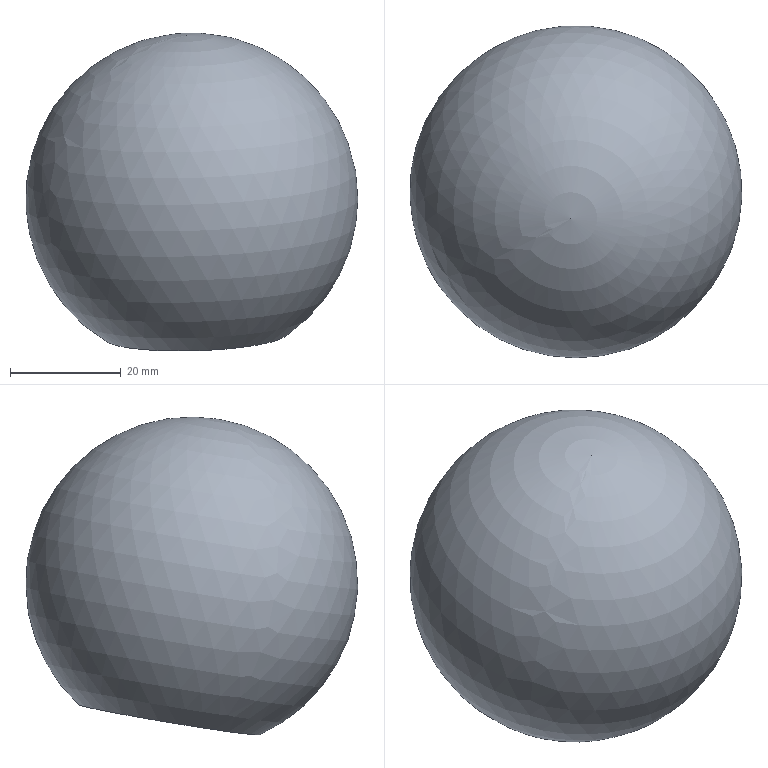Component | NX | HANDLE_KNOB | 1 solid | 5 faces | box 60 x 60 x 57.42 mm | volume 107862 mm3 | cone 2 | plane 1 | sphere 1 | cylinder 1 | commonest cylinder face diameters 14 x1
STEP:
#1=CARTESIAN_POINT('',(0.,0.,0.));
#2=DIRECTION('',(0.,0.,1.));
#3=DIRECTION('',(1.,0.,0.));
#4=AXIS2_PLACEMENT_3D('',#1,#2,#3);
#5=CARTESIAN_POINT('',(287.614,-214.929,616.056));
#6=VERTEX_POINT('',#5);
#7=CARTESIAN_POINT('',(283.581,-208.095,617.07));
#8=DIRECTION('',(-0.03071,-0.1644,0.9859));
#9=DIRECTION('',(0.5041,-0.8543,-0.1268));
#10=AXIS2_PLACEMENT_3D('',#7,#8,#9);
#11=CIRCLE('',#10,8.);
#12=CARTESIAN_POINT('',(283.581,-208.095,617.07));
#13=DIRECTION('',(-0.03071,-0.1644,0.9859));
#14=DIRECTION('',(0.5041,-0.8543,-0.1268));
#15=AXIS2_PLACEMENT_3D('',#12,#13,#14);
#16=PLANE('',#15);
#17=CARTESIAN_POINT('',(0.,0.));
#18=DIRECTION('',(1.,-0.));
#19=AXIS2_PLACEMENT_2D('',#17,#18);
#20=CIRCLE('',#19,8.);
#21=(GEOMETRIC_REPRESENTATION_CONTEXT(2)PARAMETRIC_REPRESENTATION_CONTEXT()REPRESENTATION_CONTEXT('',''));
#22=DEFINITIONAL_REPRESENTATION('',(#20),#21);
#23=PCURVE('',#16,#22);
#24=CARTESIAN_POINT('',(283.581,-208.095,617.07));
#25=DIRECTION('',(0.03071,0.1644,-0.9859));
#26=DIRECTION('',(-0.5041,0.8543,0.1268));
#27=AXIS2_PLACEMENT_3D('',#24,#25,#26);
#28=CONICAL_SURFACE('',#27,8.,0.7854);
#29=CARTESIAN_POINT('',(9.425,0.));
#30=DIRECTION('',(-1.,0.));
#31=VECTOR('',#30,1.);
#32=LINE('',#29,#31);
#33=(GEOMETRIC_REPRESENTATION_CONTEXT(2)PARAMETRIC_REPRESENTATION_CONTEXT()REPRESENTATION_CONTEXT('',''));
#34=DEFINITIONAL_REPRESENTATION('',(#32),#33);
#35=PCURVE('',#28,#34);
#36=SURFACE_CURVE('',#11,(#23,#35),.PCURVE_S1.);
#37=EDGE_CURVE('',#6,#6,#36,.T.);
#38=ORIENTED_EDGE('',*,*,#37,.T.);
#39=EDGE_LOOP('',(#38));
#40=FACE_BOUND('',#39,.T.);
#41=CARTESIAN_POINT('',(291.94,-222.262,614.968));
#42=VERTEX_POINT('',#41);
#43=CARTESIAN_POINT('',(269.268,-216.271,615.261));
#44=VERTEX_POINT('',#43);
#45=CARTESIAN_POINT('',(283.581,-208.095,617.07));
#46=DIRECTION('',(-0.03071,-0.1644,0.9859));
#47=DIRECTION('',(0.5041,-0.8543,-0.1268));
#48=AXIS2_PLACEMENT_3D('',#45,#46,#47);
#49=CIRCLE('',#48,16.583);
#50=CARTESIAN_POINT('',(0.,0.));
#51=DIRECTION('',(1.,0.));
#52=AXIS2_PLACEMENT_2D('',#50,#51);
#53=CIRCLE('',#52,16.583);
#54=(GEOMETRIC_REPRESENTATION_CONTEXT(2)PARAMETRIC_REPRESENTATION_CONTEXT()REPRESENTATION_CONTEXT('',''));
#55=DEFINITIONAL_REPRESENTATION('',(#53),#54);
#56=PCURVE('',#16,#55);
#57=CARTESIAN_POINT('',(282.813,-212.205,641.718));
#58=DIRECTION('',(-0.03071,-0.1644,0.9859));
#59=DIRECTION('',(-0.8631,-0.4931,-0.1091));
#60=AXIS2_PLACEMENT_3D('',#57,#58,#59);
#61=SPHERICAL_SURFACE('',#60,30.);
#62=CARTESIAN_POINT('',(1.571,-0.9851));
#63=CARTESIAN_POINT('',(1.666,-0.9851));
#64=CARTESIAN_POINT('',(1.856,-0.9851));
#65=CARTESIAN_POINT('',(2.142,-0.9851));
#66=CARTESIAN_POINT('',(2.428,-0.9851));
#67=CARTESIAN_POINT('',(2.713,-0.9851));
#68=CARTESIAN_POINT('',(2.999,-0.9851));
#69=CARTESIAN_POINT('',(3.284,-0.9851));
#70=CARTESIAN_POINT('',(3.57,-0.9851));
#71=CARTESIAN_POINT('',(3.856,-0.9851));
#72=CARTESIAN_POINT('',(4.141,-0.9851));
#73=CARTESIAN_POINT('',(4.427,-0.9851));
#74=CARTESIAN_POINT('',(4.712,-0.9851));
#75=CARTESIAN_POINT('',(4.998,-0.9851));
#76=CARTESIAN_POINT('',(5.284,-0.9851));
#77=CARTESIAN_POINT('',(5.569,-0.9851));
#78=CARTESIAN_POINT('',(5.855,-0.9851));
#79=CARTESIAN_POINT('',(6.14,-0.9851));
#80=CARTESIAN_POINT('',(6.426,-0.9851));
#81=CARTESIAN_POINT('',(6.712,-0.9851));
#82=CARTESIAN_POINT('',(6.997,-0.9851));
#83=CARTESIAN_POINT('',(7.283,-0.9851));
#84=CARTESIAN_POINT('',(7.568,-0.9851));
#85=CARTESIAN_POINT('',(7.759,-0.9851));
#86=CARTESIAN_POINT('',(7.854,-0.9851));
#87=B_SPLINE_CURVE_WITH_KNOTS('',3,(#62,#63,#64,#65,#66,#67,#68,#69,#70,#71,#72,#73,#74,#75,#76,#77,#78,#79,#80,#81,#82,#83,#84,#85,#86),.UNSPECIFIED.,.F.,.F.,(4,1,1,1,1,1,1,1,1,1,1,1,1,1,1,1,1,1,1,1,1,1,4),(0.,0.2856,0.5712,0.8568,1.142,1.428,1.714,1.999,2.285,2.57,2.856,3.142,3.427,3.713,3.998,4.284,4.57,4.855,5.141,5.426,5.712,5.998,6.283),.QUASI_UNIFORM_KNOTS.);
#88=(GEOMETRIC_REPRESENTATION_CONTEXT(2)PARAMETRIC_REPRESENTATION_CONTEXT()REPRESENTATION_CONTEXT('',''));
#89=DEFINITIONAL_REPRESENTATION('',(#87),#88);
#90=PCURVE('',#61,#89);
#91=SURFACE_CURVE('',#49,(#56,#90),.PCURVE_S1.);
#92=EDGE_CURVE('',#42,#44,#91,.T.);
#93=ORIENTED_EDGE('',*,*,#92,.F.);
#94=CARTESIAN_POINT('',(283.581,-208.095,617.07));
#95=DIRECTION('',(-0.03071,-0.1644,0.9859));
#96=DIRECTION('',(0.5041,-0.8543,-0.1268));
#97=AXIS2_PLACEMENT_3D('',#94,#95,#96);
#98=CIRCLE('',#97,16.583);
#99=CARTESIAN_POINT('',(0.,0.));
#100=DIRECTION('',(1.,0.));
#101=AXIS2_PLACEMENT_2D('',#99,#100);
#102=CIRCLE('',#101,16.583);
#103=(GEOMETRIC_REPRESENTATION_CONTEXT(2)PARAMETRIC_REPRESENTATION_CONTEXT()REPRESENTATION_CONTEXT('',''));
#104=DEFINITIONAL_REPRESENTATION('',(#102),#103);
#105=PCURVE('',#16,#104);
#106=CARTESIAN_POINT('',(-4.712,-0.9851));
#107=CARTESIAN_POINT('',(-4.617,-0.9851));
#108=CARTESIAN_POINT('',(-4.427,-0.9851));
#109=CARTESIAN_POINT('',(-4.141,-0.9851));
#110=CARTESIAN_POINT('',(-3.856,-0.9851));
#111=CARTESIAN_POINT('',(-3.57,-0.9851));
#112=CARTESIAN_POINT('',(-3.284,-0.9851));
#113=CARTESIAN_POINT('',(-2.999,-0.9851));
#114=CARTESIAN_POINT('',(-2.713,-0.9851));
#115=CARTESIAN_POINT('',(-2.428,-0.9851));
#116=CARTESIAN_POINT('',(-2.142,-0.9851));
#117=CARTESIAN_POINT('',(-1.856,-0.9851));
#118=CARTESIAN_POINT('',(-1.571,-0.9851));
#119=CARTESIAN_POINT('',(-1.285,-0.9851));
#120=CARTESIAN_POINT('',(-0.9996,-0.9851));
#121=CARTESIAN_POINT('',(-0.714,-0.9851));
#122=CARTESIAN_POINT('',(-0.4284,-0.9851));
#123=CARTESIAN_POINT('',(-0.1428,-0.9851));
#124=CARTESIAN_POINT('',(0.1428,-0.9851));
#125=CARTESIAN_POINT('',(0.4284,-0.9851));
#126=CARTESIAN_POINT('',(0.714,-0.9851));
#127=CARTESIAN_POINT('',(0.9996,-0.9851));
#128=CARTESIAN_POINT('',(1.285,-0.9851));
#129=CARTESIAN_POINT('',(1.476,-0.9851));
#130=CARTESIAN_POINT('',(1.571,-0.9851));
#131=B_SPLINE_CURVE_WITH_KNOTS('',3,(#106,#107,#108,#109,#110,#111,#112,#113,#114,#115,#116,#117,#118,#119,#120,#121,#122,#123,#124,#125,#126,#127,#128,#129,#130),.UNSPECIFIED.,.F.,.F.,(4,1,1,1,1,1,1,1,1,1,1,1,1,1,1,1,1,1,1,1,1,1,4),(0.,0.2856,0.5712,0.8568,1.142,1.428,1.714,1.999,2.285,2.57,2.856,3.142,3.427,3.713,3.998,4.284,4.57,4.855,5.141,5.426,5.712,5.998,6.283),.QUASI_UNIFORM_KNOTS.);
#132=(GEOMETRIC_REPRESENTATION_CONTEXT(2)PARAMETRIC_REPRESENTATION_CONTEXT()REPRESENTATION_CONTEXT('',''));
#133=DEFINITIONAL_REPRESENTATION('',(#131),#132);
#134=PCURVE('',#61,#133);
#135=SURFACE_CURVE('',#98,(#105,#134),.PCURVE_S1.);
#136=EDGE_CURVE('',#44,#42,#135,.T.);
#137=ORIENTED_EDGE('',*,*,#136,.F.);
#138=EDGE_LOOP('',(#93,#137));
#139=FACE_BOUND('',#138,.T.);
#140=ADVANCED_FACE('',(#40,#139),#16,.F.);
#141=ORIENTED_EDGE('',*,*,#92,.T.);
#142=CARTESIAN_POINT('',(281.892,-217.137,671.296));
#143=VERTEX_POINT('',#142);
#144=CARTESIAN_POINT('',(269.268,-216.271,615.261));
#145=CARTESIAN_POINT('',(262.211,-221.081,619.613));
#146=CARTESIAN_POINT('',(256.735,-225.416,627.052));
#147=CARTESIAN_POINT('',(253.936,-228.528,636.898));
#148=CARTESIAN_POINT('',(254.569,-229.774,647.81));
#149=CARTESIAN_POINT('',(258.684,-228.853,657.971));
#150=CARTESIAN_POINT('',(265.454,-226.013,665.754));
#151=CARTESIAN_POINT('',(273.619,-221.863,670.25));
#152=CARTESIAN_POINT('',(281.892,-217.137,671.296));
#153=B_SPLINE_CURVE_WITH_KNOTS('',8,(#144,#145,#146,#147,#148,#149,#150,#151,#152),.UNSPECIFIED.,.F.,.F.,(9,9),(-0.9851,1.571),.PIECEWISE_BEZIER_KNOTS.);
#154=CARTESIAN_POINT('',(6.283,0.));
#155=DIRECTION('',(0.,1.));
#156=VECTOR('',#155,1.);
#157=LINE('',#154,#156);
#158=(GEOMETRIC_REPRESENTATION_CONTEXT(2)PARAMETRIC_REPRESENTATION_CONTEXT()REPRESENTATION_CONTEXT('',''));
#159=DEFINITIONAL_REPRESENTATION('',(#157),#158);
#160=PCURVE('',#61,#159);
#161=CARTESIAN_POINT('',(0.,0.));
#162=DIRECTION('',(0.,1.));
#163=VECTOR('',#162,1.);
#164=LINE('',#161,#163);
#165=(GEOMETRIC_REPRESENTATION_CONTEXT(2)PARAMETRIC_REPRESENTATION_CONTEXT()REPRESENTATION_CONTEXT('',''));
#166=DEFINITIONAL_REPRESENTATION('',(#164),#165);
#167=PCURVE('',#61,#166);
#168=SEAM_CURVE('',#153,(#160,#167),.PCURVE_S1.);
#169=EDGE_CURVE('',#44,#143,#168,.T.);
#170=ORIENTED_EDGE('',*,*,#169,.T.);
#171=ORIENTED_EDGE('',*,*,#169,.F.);
#172=ORIENTED_EDGE('',*,*,#136,.T.);
#173=EDGE_LOOP('',(#141,#170,#171,#172));
#174=FACE_BOUND('',#173,.T.);
#175=ADVANCED_FACE('',(#174),#61,.T.);
#176=CARTESIAN_POINT('',(279.5,-205.074,635.704));
#177=VERTEX_POINT('',#176);
#178=CARTESIAN_POINT('',(286.557,-217.034,633.929));
#179=VERTEX_POINT('',#178);
#180=CARTESIAN_POINT('',(283.028,-211.054,634.817));
#181=DIRECTION('',(0.03071,0.1644,-0.9859));
#182=DIRECTION('',(0.5041,-0.8543,-0.1268));
#183=AXIS2_PLACEMENT_3D('',#180,#181,#182);
#184=CIRCLE('',#183,7.);
#185=CARTESIAN_POINT('',(283.028,-211.054,634.817));
#186=DIRECTION('',(0.03071,0.1644,-0.9859));
#187=DIRECTION('',(-0.5041,0.8543,0.1268));
#188=AXIS2_PLACEMENT_3D('',#185,#186,#187);
#189=CONICAL_SURFACE('',#188,7.,1.03);
#190=CARTESIAN_POINT('',(-3.142,0.));
#191=DIRECTION('',(1.,0.));
#192=VECTOR('',#191,1.);
#193=LINE('',#190,#192);
#194=(GEOMETRIC_REPRESENTATION_CONTEXT(2)PARAMETRIC_REPRESENTATION_CONTEXT()REPRESENTATION_CONTEXT('',''));
#195=DEFINITIONAL_REPRESENTATION('',(#193),#194);
#196=PCURVE('',#189,#195);
#197=CARTESIAN_POINT('',(283.581,-208.095,617.07));
#198=DIRECTION('',(-0.03071,-0.1644,0.9859));
#199=DIRECTION('',(0.5041,-0.8543,-0.1268));
#200=AXIS2_PLACEMENT_3D('',#197,#198,#199);
#201=CYLINDRICAL_SURFACE('',#200,7.);
#202=CARTESIAN_POINT('',(6.283,18.));
#203=DIRECTION('',(-1.,0.));
#204=VECTOR('',#203,1.);
#205=LINE('',#202,#204);
#206=(GEOMETRIC_REPRESENTATION_CONTEXT(2)PARAMETRIC_REPRESENTATION_CONTEXT()REPRESENTATION_CONTEXT('',''));
#207=DEFINITIONAL_REPRESENTATION('',(#205),#206);
#208=PCURVE('',#201,#207);
#209=SURFACE_CURVE('',#184,(#196,#208),.PCURVE_S1.);
#210=EDGE_CURVE('',#177,#179,#209,.T.);
#211=ORIENTED_EDGE('',*,*,#210,.F.);
#212=CARTESIAN_POINT('',(282.899,-211.745,638.964));
#213=VERTEX_POINT('',#212);
#214=CARTESIAN_POINT('',(282.899,-211.745,638.964));
#215=CARTESIAN_POINT('',(279.5,-205.074,635.704));
#216=B_SPLINE_CURVE_WITH_KNOTS('',1,(#214,#215),.UNSPECIFIED.,.F.,.F.,(2,2),(-8.166,0.),.PIECEWISE_BEZIER_KNOTS.);
#217=CARTESIAN_POINT('',(0.,0.));
#218=DIRECTION('',(0.,1.));
#219=VECTOR('',#218,1.);
#220=LINE('',#217,#219);
#221=(GEOMETRIC_REPRESENTATION_CONTEXT(2)PARAMETRIC_REPRESENTATION_CONTEXT()REPRESENTATION_CONTEXT('',''));
#222=DEFINITIONAL_REPRESENTATION('',(#220),#221);
#223=PCURVE('',#189,#222);
#224=CARTESIAN_POINT('',(6.283,0.));
#225=DIRECTION('',(0.,1.));
#226=VECTOR('',#225,1.);
#227=LINE('',#224,#226);
#228=(GEOMETRIC_REPRESENTATION_CONTEXT(2)PARAMETRIC_REPRESENTATION_CONTEXT()REPRESENTATION_CONTEXT('',''));
#229=DEFINITIONAL_REPRESENTATION('',(#227),#228);
#230=PCURVE('',#189,#229);
#231=SEAM_CURVE('',#216,(#223,#230),.PCURVE_S1.);
#232=EDGE_CURVE('',#213,#177,#231,.T.);
#233=ORIENTED_EDGE('',*,*,#232,.F.);
#234=ORIENTED_EDGE('',*,*,#232,.T.);
#235=CARTESIAN_POINT('',(283.028,-211.054,634.817));
#236=DIRECTION('',(0.03071,0.1644,-0.9859));
#237=DIRECTION('',(0.5041,-0.8543,-0.1268));
#238=AXIS2_PLACEMENT_3D('',#235,#236,#237);
#239=CIRCLE('',#238,7.);
#240=CARTESIAN_POINT('',(3.142,0.));
#241=DIRECTION('',(1.,0.));
#242=VECTOR('',#241,1.);
#243=LINE('',#240,#242);
#244=(GEOMETRIC_REPRESENTATION_CONTEXT(2)PARAMETRIC_REPRESENTATION_CONTEXT()REPRESENTATION_CONTEXT('',''));
#245=DEFINITIONAL_REPRESENTATION('',(#243),#244);
#246=PCURVE('',#189,#245);
#247=CARTESIAN_POINT('',(6.283,18.));
#248=DIRECTION('',(-1.,0.));
#249=VECTOR('',#248,1.);
#250=LINE('',#247,#249);
#251=(GEOMETRIC_REPRESENTATION_CONTEXT(2)PARAMETRIC_REPRESENTATION_CONTEXT()REPRESENTATION_CONTEXT('',''));
#252=DEFINITIONAL_REPRESENTATION('',(#250),#251);
#253=PCURVE('',#201,#252);
#254=SURFACE_CURVE('',#239,(#246,#253),.PCURVE_S1.);
#255=EDGE_CURVE('',#179,#177,#254,.T.);
#256=ORIENTED_EDGE('',*,*,#255,.F.);
#257=EDGE_LOOP('',(#211,#233,#234,#256));
#258=FACE_BOUND('',#257,.F.);
#259=ADVANCED_FACE('',(#258),#189,.F.);
#260=CARTESIAN_POINT('',(287.079,-214.239,617.169));
#261=VERTEX_POINT('',#260);
#262=CARTESIAN_POINT('',(283.55,-208.259,618.056));
#263=DIRECTION('',(0.03071,0.1644,-0.9859));
#264=DIRECTION('',(0.5041,-0.8543,-0.1268));
#265=AXIS2_PLACEMENT_3D('',#262,#263,#264);
#266=CIRCLE('',#265,7.);
#267=CARTESIAN_POINT('',(6.283,1.));
#268=DIRECTION('',(-1.,0.));
#269=VECTOR('',#268,1.);
#270=LINE('',#267,#269);
#271=(GEOMETRIC_REPRESENTATION_CONTEXT(2)PARAMETRIC_REPRESENTATION_CONTEXT()REPRESENTATION_CONTEXT('',''));
#272=DEFINITIONAL_REPRESENTATION('',(#270),#271);
#273=PCURVE('',#201,#272);
#274=CARTESIAN_POINT('',(3.142,-1.));
#275=DIRECTION('',(1.,0.));
#276=VECTOR('',#275,1.);
#277=LINE('',#274,#276);
#278=(GEOMETRIC_REPRESENTATION_CONTEXT(2)PARAMETRIC_REPRESENTATION_CONTEXT()REPRESENTATION_CONTEXT('',''));
#279=DEFINITIONAL_REPRESENTATION('',(#277),#278);
#280=PCURVE('',#28,#279);
#281=SURFACE_CURVE('',#266,(#273,#280),.PCURVE_S1.);
#282=EDGE_CURVE('',#261,#261,#281,.T.);
#283=ORIENTED_EDGE('',*,*,#282,.F.);
#284=CARTESIAN_POINT('',(287.079,-214.239,617.169));
#285=CARTESIAN_POINT('',(286.557,-217.034,633.929));
#286=B_SPLINE_CURVE_WITH_KNOTS('',1,(#284,#285),.UNSPECIFIED.,.F.,.F.,(2,2),(1.,18.),.PIECEWISE_BEZIER_KNOTS.);
#287=CARTESIAN_POINT('',(6.283,0.));
#288=DIRECTION('',(0.,1.));
#289=VECTOR('',#288,1.);
#290=LINE('',#287,#289);
#291=(GEOMETRIC_REPRESENTATION_CONTEXT(2)PARAMETRIC_REPRESENTATION_CONTEXT()REPRESENTATION_CONTEXT('',''));
#292=DEFINITIONAL_REPRESENTATION('',(#290),#291);
#293=PCURVE('',#201,#292);
#294=CARTESIAN_POINT('',(0.,0.));
#295=DIRECTION('',(0.,1.));
#296=VECTOR('',#295,1.);
#297=LINE('',#294,#296);
#298=(GEOMETRIC_REPRESENTATION_CONTEXT(2)PARAMETRIC_REPRESENTATION_CONTEXT()REPRESENTATION_CONTEXT('',''));
#299=DEFINITIONAL_REPRESENTATION('',(#297),#298);
#300=PCURVE('',#201,#299);
#301=SEAM_CURVE('',#286,(#293,#300),.PCURVE_S1.);
#302=EDGE_CURVE('',#261,#179,#301,.T.);
#303=ORIENTED_EDGE('',*,*,#302,.T.);
#304=ORIENTED_EDGE('',*,*,#255,.T.);
#305=ORIENTED_EDGE('',*,*,#210,.T.);
#306=ORIENTED_EDGE('',*,*,#302,.F.);
#307=EDGE_LOOP('',(#283,#303,#304,#305,#306));
#308=FACE_BOUND('',#307,.F.);
#309=ADVANCED_FACE('',(#308),#201,.F.);
#310=ORIENTED_EDGE('',*,*,#282,.T.);
#311=CARTESIAN_POINT('',(287.079,-214.239,617.169));
#312=CARTESIAN_POINT('',(287.614,-214.929,616.056));
#313=B_SPLINE_CURVE_WITH_KNOTS('',1,(#311,#312),.UNSPECIFIED.,.F.,.F.,(2,2),(-1.414,0.),.PIECEWISE_BEZIER_KNOTS.);
#314=CARTESIAN_POINT('',(9.425,0.));
#315=DIRECTION('',(0.,1.));
#316=VECTOR('',#315,1.);
#317=LINE('',#314,#316);
#318=(GEOMETRIC_REPRESENTATION_CONTEXT(2)PARAMETRIC_REPRESENTATION_CONTEXT()REPRESENTATION_CONTEXT('',''));
#319=DEFINITIONAL_REPRESENTATION('',(#317),#318);
#320=PCURVE('',#28,#319);
#321=CARTESIAN_POINT('',(3.142,0.));
#322=DIRECTION('',(0.,1.));
#323=VECTOR('',#322,1.);
#324=LINE('',#321,#323);
#325=(GEOMETRIC_REPRESENTATION_CONTEXT(2)PARAMETRIC_REPRESENTATION_CONTEXT()REPRESENTATION_CONTEXT('',''));
#326=DEFINITIONAL_REPRESENTATION('',(#324),#325);
#327=PCURVE('',#28,#326);
#328=SEAM_CURVE('',#313,(#320,#327),.PCURVE_S1.);
#329=EDGE_CURVE('',#261,#6,#328,.T.);
#330=ORIENTED_EDGE('',*,*,#329,.T.);
#331=ORIENTED_EDGE('',*,*,#37,.T.);
#332=ORIENTED_EDGE('',*,*,#329,.F.);
#333=EDGE_LOOP('',(#310,#330,#331,#332));
#334=FACE_BOUND('',#333,.F.);
#335=ADVANCED_FACE('',(#334),#28,.F.);
#336=CLOSED_SHELL('',(#140,#175,#259,#309,#335));
#337=MANIFOLD_SOLID_BREP('',#336);
#338=(LENGTH_UNIT()NAMED_UNIT(*)SI_UNIT(.MILLI.,.METRE.));
#339=UNCERTAINTY_MEASURE_WITH_UNIT(LENGTH_MEASURE(0.00001),#338,'','');
#340=(NAMED_UNIT(*)PLANE_ANGLE_UNIT()SI_UNIT($,.RADIAN.));
#341=(NAMED_UNIT(*)SI_UNIT($,.STERADIAN.)SOLID_ANGLE_UNIT());
#342=(GEOMETRIC_REPRESENTATION_CONTEXT(3)GLOBAL_UNCERTAINTY_ASSIGNED_CONTEXT((#339))GLOBAL_UNIT_ASSIGNED_CONTEXT((#338,#340,#341))REPRESENTATION_CONTEXT('',''));
#343=ADVANCED_BREP_SHAPE_REPRESENTATION('',(#4,#337),#342);